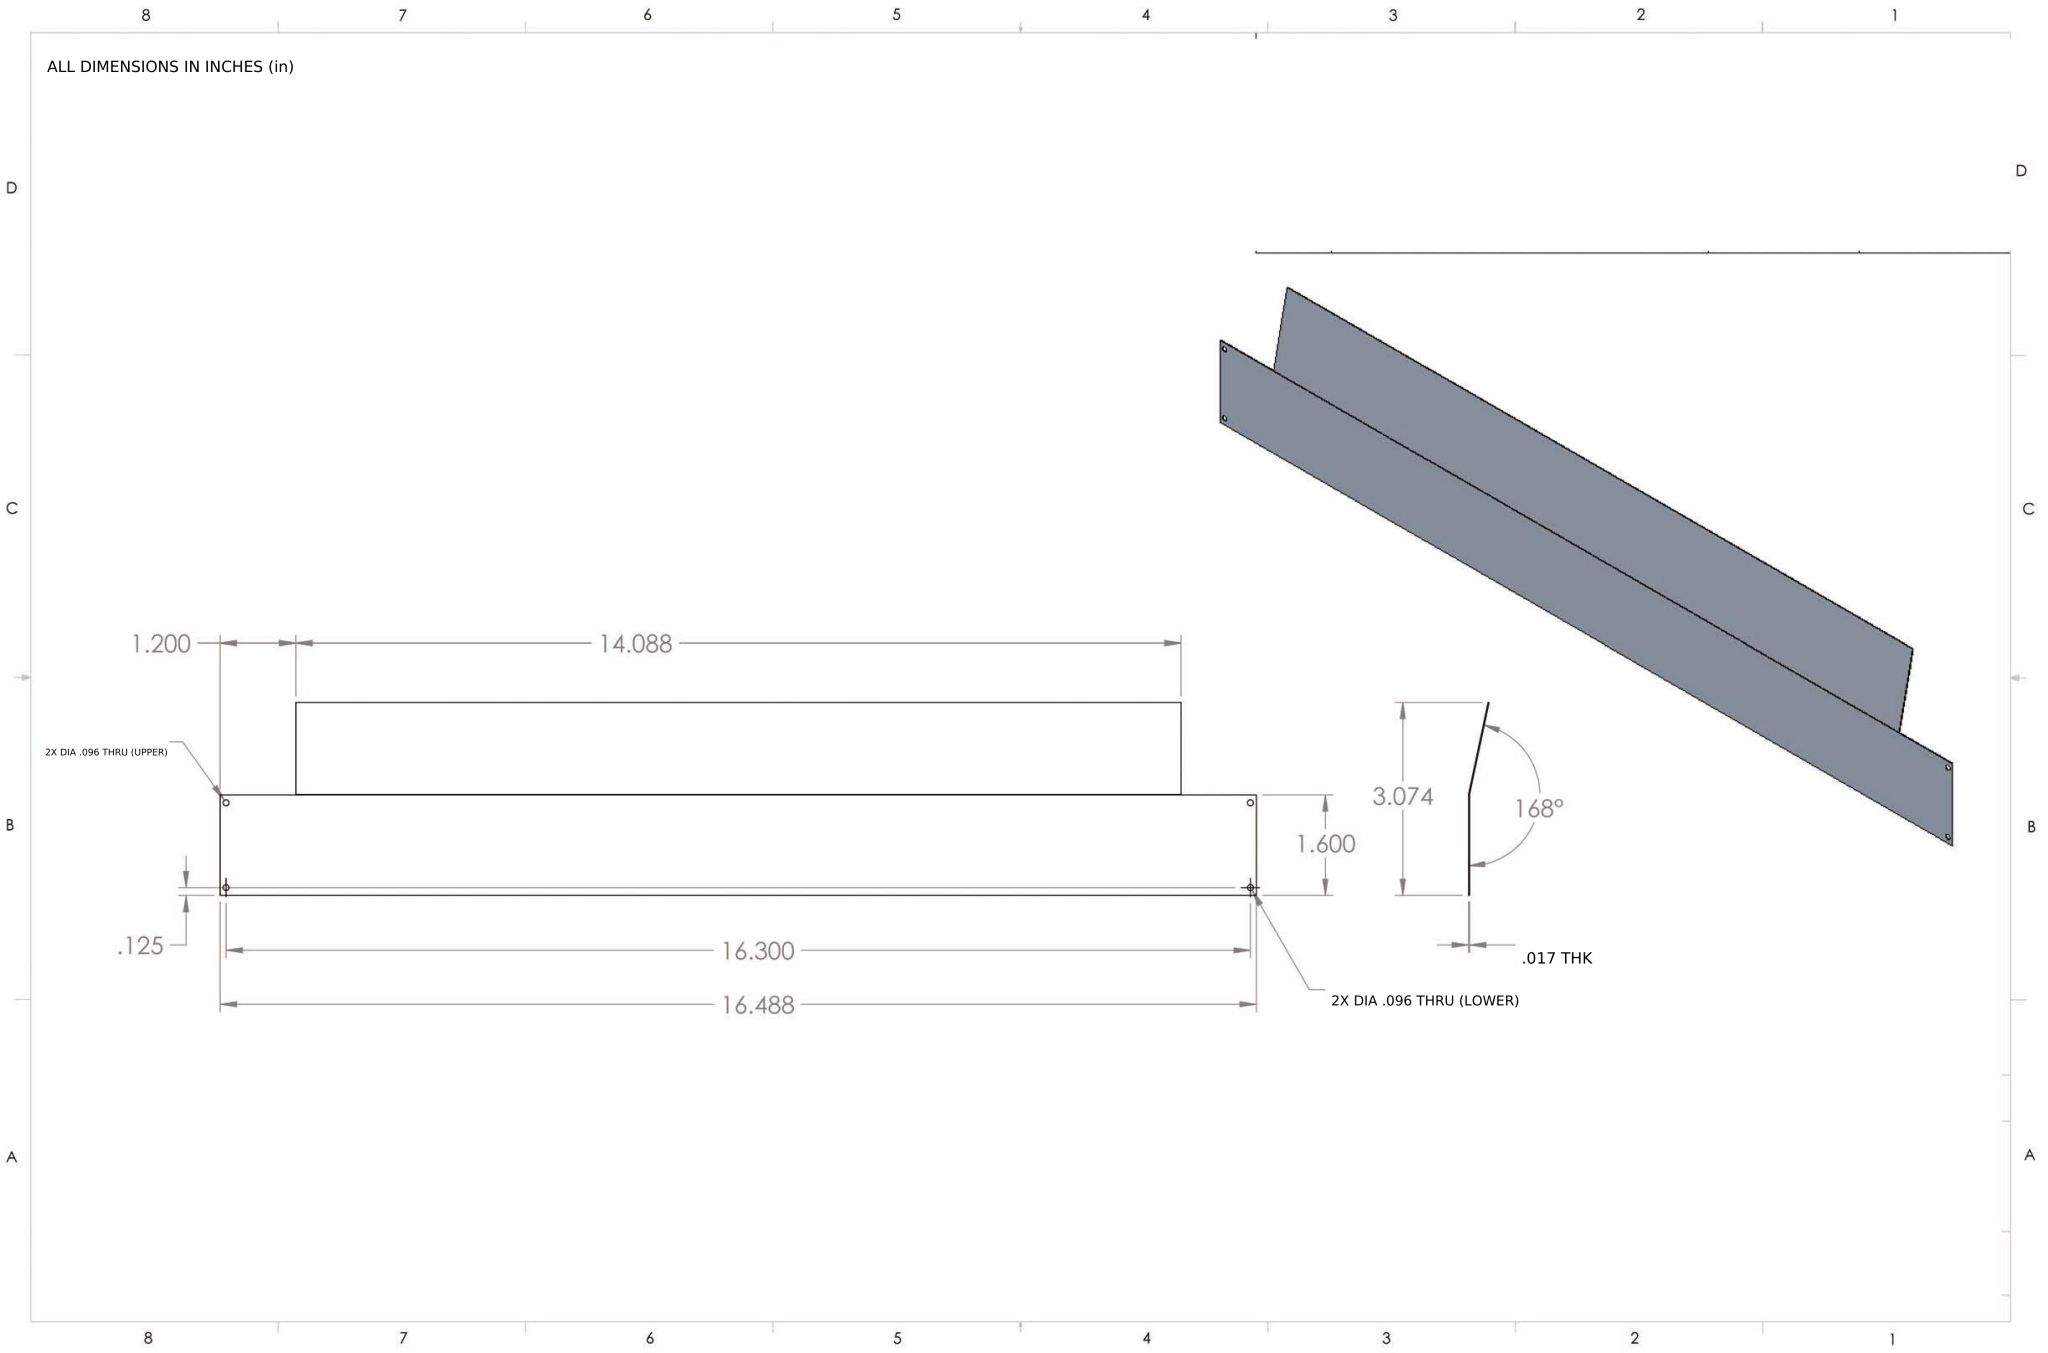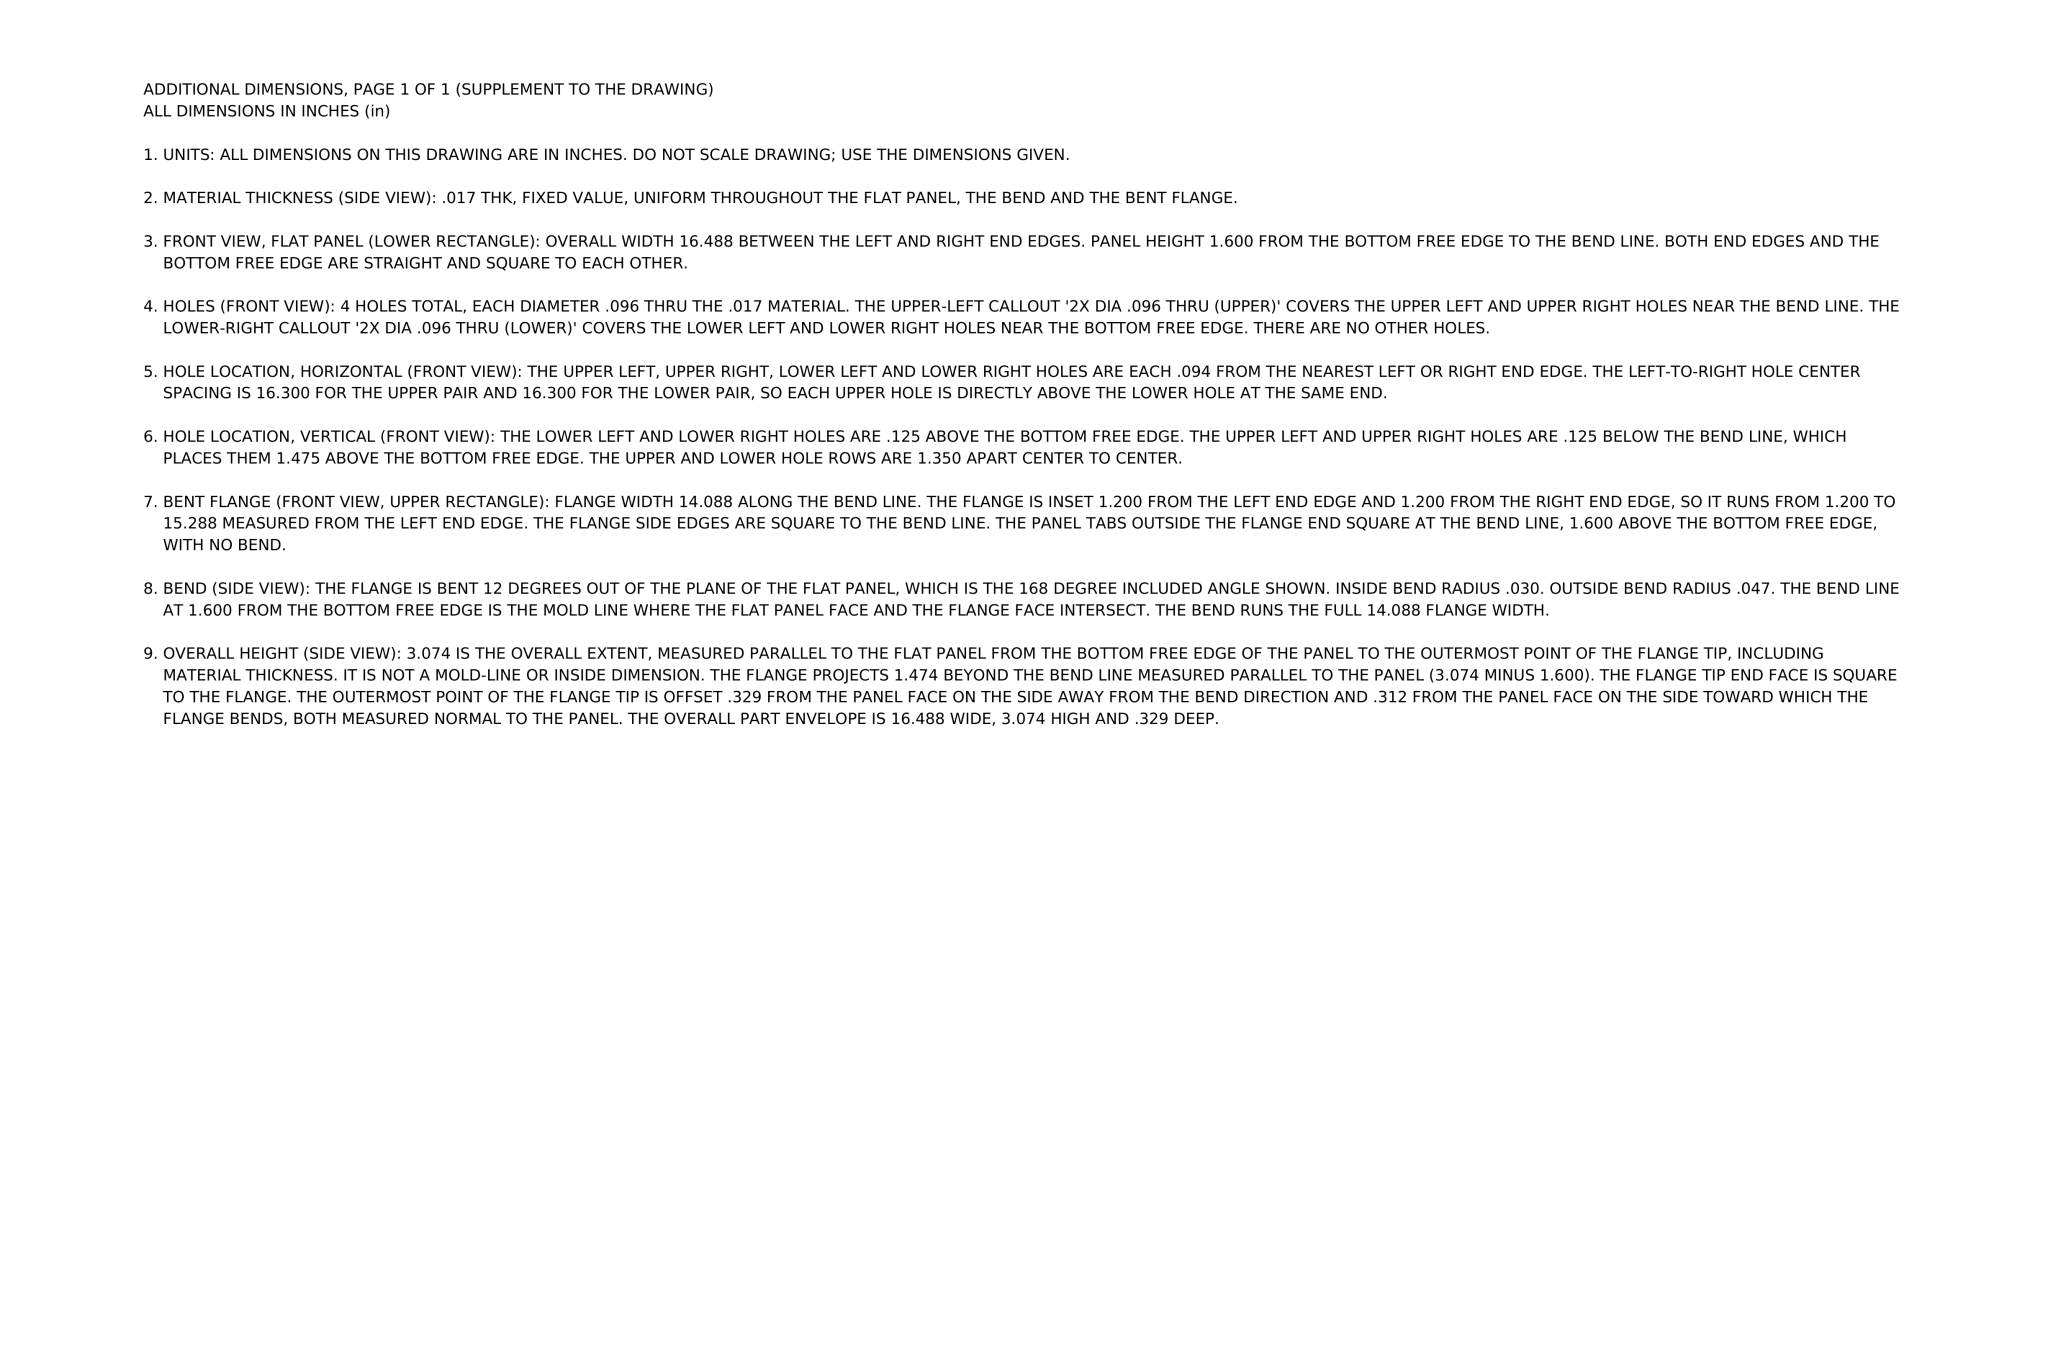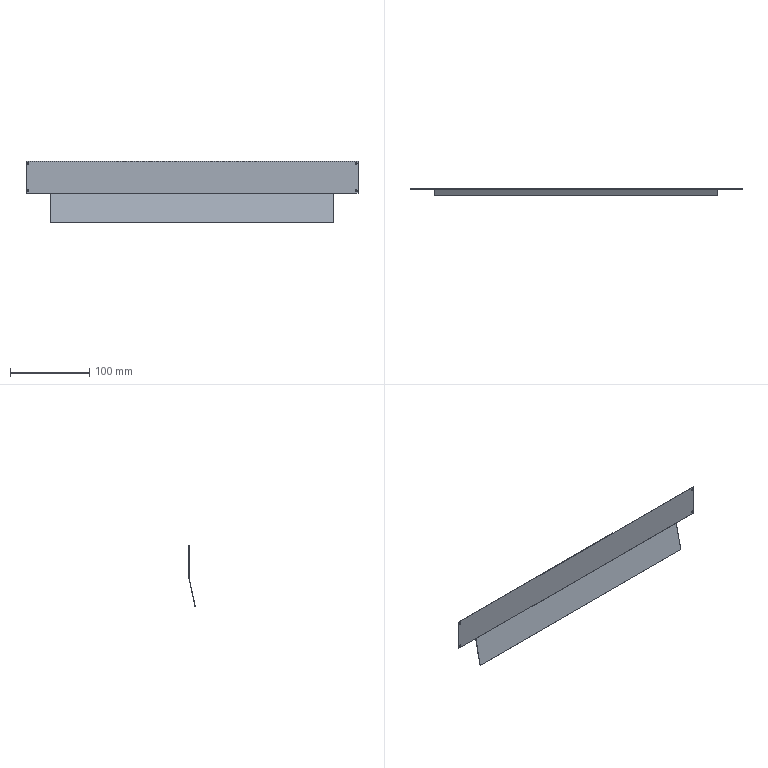Part | NX | drawing in metres | 1 solid | 24 faces | box 418.78 x 8.35 x 78.08 mm | volume 13247 mm3 | plane 14 | cylinder 10 | commonest cylinder face diameters 2.438 x8 2.388 x1 1.524 x1